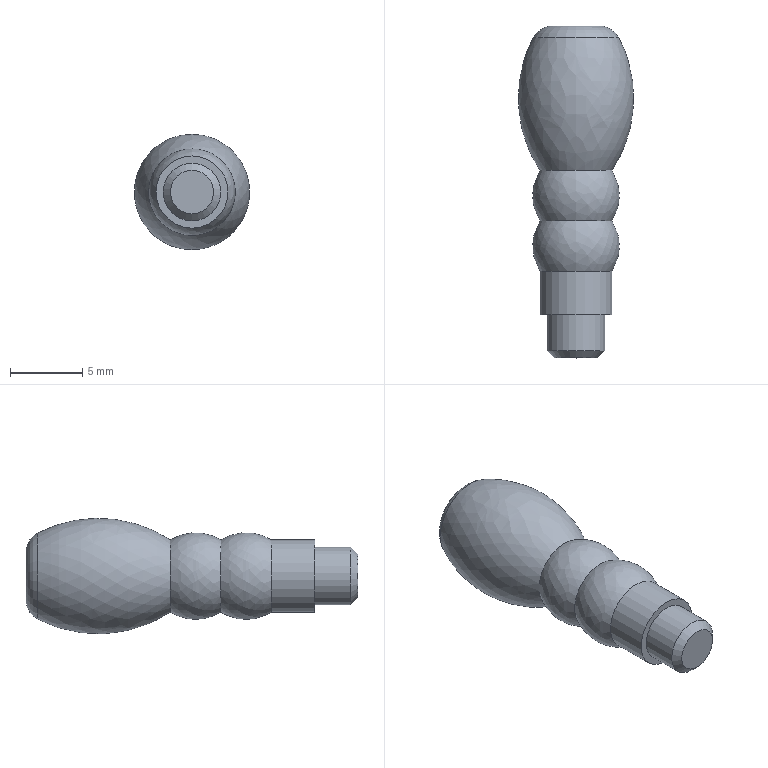Component | NX | 01 | 1 solid | 10 faces | box 8 x 23 x 8 mm | volume 666 mm3 | plane 3 | spline 3 | cylinder 2 | torus 1 | cone 1 | commonest cylinder face diameters 5 x1 4 x1
STEP:
#1=CARTESIAN_POINT('',(0.,0.,0.));
#2=DIRECTION('',(0.,0.,1.));
#3=DIRECTION('',(1.,0.,0.));
#4=AXIS2_PLACEMENT_3D('',#1,#2,#3);
#5=CARTESIAN_POINT('',(0.,-20.,-2.));
#6=VERTEX_POINT('',#5);
#7=CARTESIAN_POINT('',(0.,-20.,0.));
#8=DIRECTION('',(0.,-1.,0.));
#9=DIRECTION('',(0.,0.,-1.));
#10=AXIS2_PLACEMENT_3D('',#7,#8,#9);
#11=CIRCLE('',#10,2.);
#12=CARTESIAN_POINT('',(2.5,-20.,0.));
#13=DIRECTION('',(0.,-1.,0.));
#14=DIRECTION('',(0.,0.,-1.));
#15=AXIS2_PLACEMENT_3D('',#12,#13,#14);
#16=PLANE('',#15);
#17=CARTESIAN_POINT('',(0.,-2.5));
#18=DIRECTION('',(1.,0.));
#19=AXIS2_PLACEMENT_2D('',#17,#18);
#20=CIRCLE('',#19,2.);
#21=(GEOMETRIC_REPRESENTATION_CONTEXT(2)PARAMETRIC_REPRESENTATION_CONTEXT()REPRESENTATION_CONTEXT('',''));
#22=DEFINITIONAL_REPRESENTATION('',(#20),#21);
#23=PCURVE('',#16,#22);
#24=CARTESIAN_POINT('',(0.,-20.,0.));
#25=DIRECTION('',(0.,-1.,0.));
#26=DIRECTION('',(1.,0.,0.));
#27=AXIS2_PLACEMENT_3D('',#24,#25,#26);
#28=CYLINDRICAL_SURFACE('',#27,2.);
#29=CARTESIAN_POINT('',(4.712,0.));
#30=DIRECTION('',(1.,0.));
#31=VECTOR('',#30,1.);
#32=LINE('',#29,#31);
#33=(GEOMETRIC_REPRESENTATION_CONTEXT(2)PARAMETRIC_REPRESENTATION_CONTEXT()REPRESENTATION_CONTEXT('',''));
#34=DEFINITIONAL_REPRESENTATION('',(#32),#33);
#35=PCURVE('',#28,#34);
#36=SURFACE_CURVE('',#11,(#23,#35),.PCURVE_S1.);
#37=EDGE_CURVE('',#6,#6,#36,.T.);
#38=ORIENTED_EDGE('',*,*,#37,.F.);
#39=EDGE_LOOP('',(#38));
#40=FACE_BOUND('',#39,.T.);
#41=CARTESIAN_POINT('',(0.,-20.,2.5));
#42=VERTEX_POINT('',#41);
#43=CARTESIAN_POINT('',(0.,-20.,0.));
#44=DIRECTION('',(0.,1.,0.));
#45=DIRECTION('',(0.,0.,1.));
#46=AXIS2_PLACEMENT_3D('',#43,#44,#45);
#47=CIRCLE('',#46,2.5);
#48=CARTESIAN_POINT('',(-2.5,-2.5));
#49=CARTESIAN_POINT('',(-2.5,1.83));
#50=CARTESIAN_POINT('',(1.25,-0.3349));
#51=CARTESIAN_POINT('',(5.,-2.5));
#52=CARTESIAN_POINT('',(1.25,-4.665));
#53=CARTESIAN_POINT('',(-2.5,-6.83));
#54=CARTESIAN_POINT('',(-2.5,-2.5));
#55=(BOUNDED_CURVE()B_SPLINE_CURVE(2,(#48,#49,#50,#51,#52,#53,#54),.UNSPECIFIED.,.T.,.F.)B_SPLINE_CURVE_WITH_KNOTS((1,2,2,2,2,1),(-2.094,0.,2.094,4.189,6.283,8.378),.UNSPECIFIED.)CURVE()GEOMETRIC_REPRESENTATION_ITEM()RATIONAL_B_SPLINE_CURVE((1.,0.5,1.,0.5,1.,0.5,1.))REPRESENTATION_ITEM(''));
#56=(GEOMETRIC_REPRESENTATION_CONTEXT(2)PARAMETRIC_REPRESENTATION_CONTEXT()REPRESENTATION_CONTEXT('',''));
#57=DEFINITIONAL_REPRESENTATION('',(#55),#56);
#58=PCURVE('',#16,#57);
#59=CARTESIAN_POINT('',(0.,0.,0.));
#60=DIRECTION('',(0.,1.,0.));
#61=DIRECTION('',(0.,0.,1.));
#62=AXIS2_PLACEMENT_3D('',#59,#60,#61);
#63=CYLINDRICAL_SURFACE('',#62,2.5);
#64=CARTESIAN_POINT('',(0.,-20.));
#65=DIRECTION('',(1.,0.));
#66=VECTOR('',#65,1.);
#67=LINE('',#64,#66);
#68=(GEOMETRIC_REPRESENTATION_CONTEXT(2)PARAMETRIC_REPRESENTATION_CONTEXT()REPRESENTATION_CONTEXT('',''));
#69=DEFINITIONAL_REPRESENTATION('',(#67),#68);
#70=PCURVE('',#63,#69);
#71=SURFACE_CURVE('',#47,(#58,#70),.PCURVE_S1.);
#72=EDGE_CURVE('',#42,#42,#71,.T.);
#73=ORIENTED_EDGE('',*,*,#72,.F.);
#74=EDGE_LOOP('',(#73));
#75=FACE_BOUND('',#74,.T.);
#76=ADVANCED_FACE('',(#40,#75),#16,.T.);
#77=ORIENTED_EDGE('',*,*,#72,.T.);
#78=CARTESIAN_POINT('',(0.,-17.,2.5));
#79=VERTEX_POINT('',#78);
#80=CARTESIAN_POINT('',(0.,-20.,2.5));
#81=CARTESIAN_POINT('',(0.,-17.,2.5));
#82=B_SPLINE_CURVE_WITH_KNOTS('',1,(#80,#81),.UNSPECIFIED.,.F.,.F.,(2,2),(-20.,-17.),.PIECEWISE_BEZIER_KNOTS.);
#83=CARTESIAN_POINT('',(6.283,0.));
#84=DIRECTION('',(0.,1.));
#85=VECTOR('',#84,1.);
#86=LINE('',#83,#85);
#87=(GEOMETRIC_REPRESENTATION_CONTEXT(2)PARAMETRIC_REPRESENTATION_CONTEXT()REPRESENTATION_CONTEXT('',''));
#88=DEFINITIONAL_REPRESENTATION('',(#86),#87);
#89=PCURVE('',#63,#88);
#90=CARTESIAN_POINT('',(0.,0.));
#91=DIRECTION('',(0.,1.));
#92=VECTOR('',#91,1.);
#93=LINE('',#90,#92);
#94=(GEOMETRIC_REPRESENTATION_CONTEXT(2)PARAMETRIC_REPRESENTATION_CONTEXT()REPRESENTATION_CONTEXT('',''));
#95=DEFINITIONAL_REPRESENTATION('',(#93),#94);
#96=PCURVE('',#63,#95);
#97=SEAM_CURVE('',#82,(#89,#96),.PCURVE_S1.);
#98=EDGE_CURVE('',#42,#79,#97,.T.);
#99=ORIENTED_EDGE('',*,*,#98,.T.);
#100=CARTESIAN_POINT('',(0.,-17.,0.));
#101=DIRECTION('',(0.,1.,0.));
#102=DIRECTION('',(0.,0.,1.));
#103=AXIS2_PLACEMENT_3D('',#100,#101,#102);
#104=CIRCLE('',#103,2.5);
#105=CARTESIAN_POINT('',(0.,-17.));
#106=DIRECTION('',(1.,0.));
#107=VECTOR('',#106,1.);
#108=LINE('',#105,#107);
#109=(GEOMETRIC_REPRESENTATION_CONTEXT(2)PARAMETRIC_REPRESENTATION_CONTEXT()REPRESENTATION_CONTEXT('',''));
#110=DEFINITIONAL_REPRESENTATION('',(#108),#109);
#111=PCURVE('',#63,#110);
#112=CARTESIAN_POINT('',(0.,-13.5,2.5));
#113=CARTESIAN_POINT('',(5.,-13.5,2.5));
#114=CARTESIAN_POINT('',(5.,-13.5,-2.5));
#115=CARTESIAN_POINT('',(0.,-13.5,-2.5));
#116=CARTESIAN_POINT('',(-5.,-13.5,-2.5));
#117=CARTESIAN_POINT('',(-5.,-13.5,2.5));
#118=CARTESIAN_POINT('',(0.,-13.5,2.5));
#119=CARTESIAN_POINT('',(0.,-14.601,3.185));
#120=CARTESIAN_POINT('',(6.371,-14.601,3.185));
#121=CARTESIAN_POINT('',(6.371,-14.601,-3.185));
#122=CARTESIAN_POINT('',(0.,-14.601,-3.185));
#123=CARTESIAN_POINT('',(-6.371,-14.601,-3.185));
#124=CARTESIAN_POINT('',(-6.371,-14.601,3.185));
#125=CARTESIAN_POINT('',(0.,-14.601,3.185));
#126=CARTESIAN_POINT('',(0.,-15.899,3.185));
#127=CARTESIAN_POINT('',(6.371,-15.899,3.185));
#128=CARTESIAN_POINT('',(6.371,-15.899,-3.185));
#129=CARTESIAN_POINT('',(0.,-15.899,-3.185));
#130=CARTESIAN_POINT('',(-6.371,-15.899,-3.185));
#131=CARTESIAN_POINT('',(-6.371,-15.899,3.185));
#132=CARTESIAN_POINT('',(0.,-15.899,3.185));
#133=CARTESIAN_POINT('',(0.,-17.,2.5));
#134=CARTESIAN_POINT('',(5.,-17.,2.5));
#135=CARTESIAN_POINT('',(5.,-17.,-2.5));
#136=CARTESIAN_POINT('',(0.,-17.,-2.5));
#137=CARTESIAN_POINT('',(-5.,-17.,-2.5));
#138=CARTESIAN_POINT('',(-5.,-17.,2.5));
#139=CARTESIAN_POINT('',(0.,-17.,2.5));
#140=(BOUNDED_SURFACE()B_SPLINE_SURFACE(3,3,((#112,#113,#114,#115,#116,#117,#118),(#119,#120,#121,#122,#123,#124,#125),(#126,#127,#128,#129,#130,#131,#132),(#133,#134,#135,#136,#137,#138,#139)),.UNSPECIFIED.,.F.,.T.,.F.)B_SPLINE_SURFACE_WITH_KNOTS((4,4),(1,3,3,3,1),(0.,1.),(-0.5,0.,0.5,1.,1.5),.UNSPECIFIED.)GEOMETRIC_REPRESENTATION_ITEM()RATIONAL_B_SPLINE_SURFACE(((1.,0.3333,0.3333,1.,0.3333,0.3333,1.),(0.8994,0.2998,0.2998,0.8994,0.2998,0.2998,0.8994),(0.8994,0.2998,0.2998,0.8994,0.2998,0.2998,0.8994),(1.,0.3333,0.3333,1.,0.3333,0.3333,1.)))REPRESENTATION_ITEM('')SURFACE());
#141=CARTESIAN_POINT('',(1.,0.));
#142=CARTESIAN_POINT('',(1.,0.02352));
#143=CARTESIAN_POINT('',(1.,0.06491));
#144=CARTESIAN_POINT('',(1.,0.1146));
#145=CARTESIAN_POINT('',(1.,0.1575));
#146=CARTESIAN_POINT('',(1.,0.196));
#147=CARTESIAN_POINT('',(1.,0.2322));
#148=CARTESIAN_POINT('',(1.,0.2678));
#149=CARTESIAN_POINT('',(1.,0.304));
#150=CARTESIAN_POINT('',(1.,0.3425));
#151=CARTESIAN_POINT('',(1.,0.3856));
#152=CARTESIAN_POINT('',(1.,0.4343));
#153=CARTESIAN_POINT('',(1.,0.5));
#154=CARTESIAN_POINT('',(1.,0.5657));
#155=CARTESIAN_POINT('',(1.,0.6144));
#156=CARTESIAN_POINT('',(1.,0.6575));
#157=CARTESIAN_POINT('',(1.,0.696));
#158=CARTESIAN_POINT('',(1.,0.7322));
#159=CARTESIAN_POINT('',(1.,0.7678));
#160=CARTESIAN_POINT('',(1.,0.804));
#161=CARTESIAN_POINT('',(1.,0.8425));
#162=CARTESIAN_POINT('',(1.,0.8854));
#163=CARTESIAN_POINT('',(1.,0.9351));
#164=CARTESIAN_POINT('',(1.,0.9765));
#165=CARTESIAN_POINT('',(1.,1.));
#166=B_SPLINE_CURVE_WITH_KNOTS('',3,(#141,#142,#143,#144,#145,#146,#147,#148,#149,#150,#151,#152,#153,#154,#155,#156,#157,#158,#159,#160,#161,#162,#163,#164,#165),.UNSPECIFIED.,.F.,.F.,(4,1,1,1,1,1,1,1,1,1,1,1,1,1,1,1,1,1,1,1,1,1,4),(0.,0.2856,0.5712,0.8568,1.142,1.428,1.714,1.999,2.285,2.57,2.856,3.142,3.427,3.713,3.998,4.284,4.57,4.855,5.141,5.426,5.712,5.998,6.283),.QUASI_UNIFORM_KNOTS.);
#167=(GEOMETRIC_REPRESENTATION_CONTEXT(2)PARAMETRIC_REPRESENTATION_CONTEXT()REPRESENTATION_CONTEXT('',''));
#168=DEFINITIONAL_REPRESENTATION('',(#166),#167);
#169=PCURVE('',#140,#168);
#170=SURFACE_CURVE('',#104,(#111,#169),.PCURVE_S1.);
#171=EDGE_CURVE('',#79,#79,#170,.T.);
#172=ORIENTED_EDGE('',*,*,#171,.F.);
#173=ORIENTED_EDGE('',*,*,#98,.F.);
#174=EDGE_LOOP('',(#77,#99,#172,#173));
#175=FACE_BOUND('',#174,.T.);
#176=ADVANCED_FACE('',(#175),#63,.T.);
#177=ORIENTED_EDGE('',*,*,#171,.T.);
#178=CARTESIAN_POINT('',(0.,-13.5,2.5));
#179=VERTEX_POINT('',#178);
#180=CARTESIAN_POINT('',(0.,-13.5,2.5));
#181=CARTESIAN_POINT('',(0.,-14.601,3.185));
#182=CARTESIAN_POINT('',(0.,-15.899,3.185));
#183=CARTESIAN_POINT('',(0.,-17.,2.5));
#184=(BOUNDED_CURVE()B_SPLINE_CURVE(3,(#180,#181,#182,#183),.UNSPECIFIED.,.F.,.F.)B_SPLINE_CURVE_WITH_KNOTS((4,4),(0.,1.),.PIECEWISE_BEZIER_KNOTS.)CURVE()GEOMETRIC_REPRESENTATION_ITEM()RATIONAL_B_SPLINE_CURVE((1.,0.8994,0.8994,1.))REPRESENTATION_ITEM(''));
#185=CARTESIAN_POINT('',(0.,1.));
#186=DIRECTION('',(1.,0.));
#187=VECTOR('',#186,1.);
#188=LINE('',#185,#187);
#189=(GEOMETRIC_REPRESENTATION_CONTEXT(2)PARAMETRIC_REPRESENTATION_CONTEXT()REPRESENTATION_CONTEXT('',''));
#190=DEFINITIONAL_REPRESENTATION('',(#188),#189);
#191=PCURVE('',#140,#190);
#192=CARTESIAN_POINT('',(0.,0.));
#193=DIRECTION('',(1.,0.));
#194=VECTOR('',#193,1.);
#195=LINE('',#192,#194);
#196=(GEOMETRIC_REPRESENTATION_CONTEXT(2)PARAMETRIC_REPRESENTATION_CONTEXT()REPRESENTATION_CONTEXT('',''));
#197=DEFINITIONAL_REPRESENTATION('',(#195),#196);
#198=PCURVE('',#140,#197);
#199=SEAM_CURVE('',#184,(#191,#198),.PCURVE_S1.);
#200=EDGE_CURVE('',#179,#79,#199,.T.);
#201=ORIENTED_EDGE('',*,*,#200,.F.);
#202=CARTESIAN_POINT('',(0.,-13.5,0.));
#203=DIRECTION('',(0.,1.,0.));
#204=DIRECTION('',(0.,0.,1.));
#205=AXIS2_PLACEMENT_3D('',#202,#203,#204);
#206=CIRCLE('',#205,2.5);
#207=CARTESIAN_POINT('',(0.,0.));
#208=CARTESIAN_POINT('',(0.,0.02352));
#209=CARTESIAN_POINT('',(0.,0.06491));
#210=CARTESIAN_POINT('',(0.,0.1146));
#211=CARTESIAN_POINT('',(0.,0.1575));
#212=CARTESIAN_POINT('',(0.,0.196));
#213=CARTESIAN_POINT('',(0.,0.2322));
#214=CARTESIAN_POINT('',(0.,0.2678));
#215=CARTESIAN_POINT('',(0.,0.304));
#216=CARTESIAN_POINT('',(0.,0.3425));
#217=CARTESIAN_POINT('',(0.,0.3856));
#218=CARTESIAN_POINT('',(0.,0.4343));
#219=CARTESIAN_POINT('',(0.,0.5));
#220=CARTESIAN_POINT('',(0.,0.5657));
#221=CARTESIAN_POINT('',(0.,0.6144));
#222=CARTESIAN_POINT('',(0.,0.6575));
#223=CARTESIAN_POINT('',(0.,0.696));
#224=CARTESIAN_POINT('',(0.,0.7322));
#225=CARTESIAN_POINT('',(0.,0.7678));
#226=CARTESIAN_POINT('',(0.,0.804));
#227=CARTESIAN_POINT('',(0.,0.8425));
#228=CARTESIAN_POINT('',(0.,0.8854));
#229=CARTESIAN_POINT('',(0.,0.9351));
#230=CARTESIAN_POINT('',(0.,0.9765));
#231=CARTESIAN_POINT('',(0.,1.));
#232=B_SPLINE_CURVE_WITH_KNOTS('',3,(#207,#208,#209,#210,#211,#212,#213,#214,#215,#216,#217,#218,#219,#220,#221,#222,#223,#224,#225,#226,#227,#228,#229,#230,#231),.UNSPECIFIED.,.F.,.F.,(4,1,1,1,1,1,1,1,1,1,1,1,1,1,1,1,1,1,1,1,1,1,4),(0.,0.2856,0.5712,0.8568,1.142,1.428,1.714,1.999,2.285,2.57,2.856,3.142,3.427,3.713,3.998,4.284,4.57,4.855,5.141,5.426,5.712,5.998,6.283),.QUASI_UNIFORM_KNOTS.);
#233=(GEOMETRIC_REPRESENTATION_CONTEXT(2)PARAMETRIC_REPRESENTATION_CONTEXT()REPRESENTATION_CONTEXT('',''));
#234=DEFINITIONAL_REPRESENTATION('',(#232),#233);
#235=PCURVE('',#140,#234);
#236=CARTESIAN_POINT('',(0.,-10.,2.5));
#237=CARTESIAN_POINT('',(5.,-10.,2.5));
#238=CARTESIAN_POINT('',(5.,-10.,-2.5));
#239=CARTESIAN_POINT('',(0.,-10.,-2.5));
#240=CARTESIAN_POINT('',(-5.,-10.,-2.5));
#241=CARTESIAN_POINT('',(-5.,-10.,2.5));
#242=CARTESIAN_POINT('',(0.,-10.,2.5));
#243=CARTESIAN_POINT('',(0.,-11.101,3.185));
#244=CARTESIAN_POINT('',(6.371,-11.101,3.185));
#245=CARTESIAN_POINT('',(6.371,-11.101,-3.185));
#246=CARTESIAN_POINT('',(0.,-11.101,-3.185));
#247=CARTESIAN_POINT('',(-6.371,-11.101,-3.185));
#248=CARTESIAN_POINT('',(-6.371,-11.101,3.185));
#249=CARTESIAN_POINT('',(0.,-11.101,3.185));
#250=CARTESIAN_POINT('',(0.,-12.399,3.185));
#251=CARTESIAN_POINT('',(6.371,-12.399,3.185));
#252=CARTESIAN_POINT('',(6.371,-12.399,-3.185));
#253=CARTESIAN_POINT('',(0.,-12.399,-3.185));
#254=CARTESIAN_POINT('',(-6.371,-12.399,-3.185));
#255=CARTESIAN_POINT('',(-6.371,-12.399,3.185));
#256=CARTESIAN_POINT('',(0.,-12.399,3.185));
#257=CARTESIAN_POINT('',(0.,-13.5,2.5));
#258=CARTESIAN_POINT('',(5.,-13.5,2.5));
#259=CARTESIAN_POINT('',(5.,-13.5,-2.5));
#260=CARTESIAN_POINT('',(0.,-13.5,-2.5));
#261=CARTESIAN_POINT('',(-5.,-13.5,-2.5));
#262=CARTESIAN_POINT('',(-5.,-13.5,2.5));
#263=CARTESIAN_POINT('',(0.,-13.5,2.5));
#264=(BOUNDED_SURFACE()B_SPLINE_SURFACE(3,3,((#236,#237,#238,#239,#240,#241,#242),(#243,#244,#245,#246,#247,#248,#249),(#250,#251,#252,#253,#254,#255,#256),(#257,#258,#259,#260,#261,#262,#263)),.UNSPECIFIED.,.F.,.T.,.F.)B_SPLINE_SURFACE_WITH_KNOTS((4,4),(1,3,3,3,1),(0.,1.),(-0.5,0.,0.5,1.,1.5),.UNSPECIFIED.)GEOMETRIC_REPRESENTATION_ITEM()RATIONAL_B_SPLINE_SURFACE(((1.,0.3333,0.3333,1.,0.3333,0.3333,1.),(0.8994,0.2998,0.2998,0.8994,0.2998,0.2998,0.8994),(0.8994,0.2998,0.2998,0.8994,0.2998,0.2998,0.8994),(1.,0.3333,0.3333,1.,0.3333,0.3333,1.)))REPRESENTATION_ITEM('')SURFACE());
#265=CARTESIAN_POINT('',(1.,0.));
#266=CARTESIAN_POINT('',(1.,0.02352));
#267=CARTESIAN_POINT('',(1.,0.06491));
#268=CARTESIAN_POINT('',(1.,0.1146));
#269=CARTESIAN_POINT('',(1.,0.1575));
#270=CARTESIAN_POINT('',(1.,0.196));
#271=CARTESIAN_POINT('',(1.,0.2322));
#272=CARTESIAN_POINT('',(1.,0.2678));
#273=CARTESIAN_POINT('',(1.,0.304));
#274=CARTESIAN_POINT('',(1.,0.3425));
#275=CARTESIAN_POINT('',(1.,0.3856));
#276=CARTESIAN_POINT('',(1.,0.4343));
#277=CARTESIAN_POINT('',(1.,0.5));
#278=CARTESIAN_POINT('',(1.,0.5657));
#279=CARTESIAN_POINT('',(1.,0.6144));
#280=CARTESIAN_POINT('',(1.,0.6575));
#281=CARTESIAN_POINT('',(1.,0.696));
#282=CARTESIAN_POINT('',(1.,0.7322));
#283=CARTESIAN_POINT('',(1.,0.7678));
#284=CARTESIAN_POINT('',(1.,0.804));
#285=CARTESIAN_POINT('',(1.,0.8425));
#286=CARTESIAN_POINT('',(1.,0.8854));
#287=CARTESIAN_POINT('',(1.,0.9351));
#288=CARTESIAN_POINT('',(1.,0.9765));
#289=CARTESIAN_POINT('',(1.,1.));
#290=B_SPLINE_CURVE_WITH_KNOTS('',3,(#265,#266,#267,#268,#269,#270,#271,#272,#273,#274,#275,#276,#277,#278,#279,#280,#281,#282,#283,#284,#285,#286,#287,#288,#289),.UNSPECIFIED.,.F.,.F.,(4,1,1,1,1,1,1,1,1,1,1,1,1,1,1,1,1,1,1,1,1,1,4),(0.,0.2856,0.5712,0.8568,1.142,1.428,1.714,1.999,2.285,2.57,2.856,3.142,3.427,3.713,3.998,4.284,4.57,4.855,5.141,5.426,5.712,5.998,6.283),.QUASI_UNIFORM_KNOTS.);
#291=(GEOMETRIC_REPRESENTATION_CONTEXT(2)PARAMETRIC_REPRESENTATION_CONTEXT()REPRESENTATION_CONTEXT('',''));
#292=DEFINITIONAL_REPRESENTATION('',(#290),#291);
#293=PCURVE('',#264,#292);
#294=SURFACE_CURVE('',#206,(#235,#293),.PCURVE_S1.);
#295=EDGE_CURVE('',#179,#179,#294,.T.);
#296=ORIENTED_EDGE('',*,*,#295,.F.);
#297=ORIENTED_EDGE('',*,*,#200,.T.);
#298=EDGE_LOOP('',(#177,#201,#296,#297));
#299=FACE_BOUND('',#298,.T.);
#300=ADVANCED_FACE('',(#299),#140,.T.);
#301=ORIENTED_EDGE('',*,*,#295,.T.);
#302=CARTESIAN_POINT('',(0.,-10.,2.5));
#303=VERTEX_POINT('',#302);
#304=CARTESIAN_POINT('',(0.,-10.,2.5));
#305=CARTESIAN_POINT('',(0.,-11.101,3.185));
#306=CARTESIAN_POINT('',(0.,-12.399,3.185));
#307=CARTESIAN_POINT('',(0.,-13.5,2.5));
#308=(BOUNDED_CURVE()B_SPLINE_CURVE(3,(#304,#305,#306,#307),.UNSPECIFIED.,.F.,.F.)B_SPLINE_CURVE_WITH_KNOTS((4,4),(0.,1.),.PIECEWISE_BEZIER_KNOTS.)CURVE()GEOMETRIC_REPRESENTATION_ITEM()RATIONAL_B_SPLINE_CURVE((1.,0.8994,0.8994,1.))REPRESENTATION_ITEM(''));
#309=CARTESIAN_POINT('',(0.,1.));
#310=DIRECTION('',(1.,0.));
#311=VECTOR('',#310,1.);
#312=LINE('',#309,#311);
#313=(GEOMETRIC_REPRESENTATION_CONTEXT(2)PARAMETRIC_REPRESENTATION_CONTEXT()REPRESENTATION_CONTEXT('',''));
#314=DEFINITIONAL_REPRESENTATION('',(#312),#313);
#315=PCURVE('',#264,#314);
#316=CARTESIAN_POINT('',(0.,0.));
#317=DIRECTION('',(1.,0.));
#318=VECTOR('',#317,1.);
#319=LINE('',#316,#318);
#320=(GEOMETRIC_REPRESENTATION_CONTEXT(2)PARAMETRIC_REPRESENTATION_CONTEXT()REPRESENTATION_CONTEXT('',''));
#321=DEFINITIONAL_REPRESENTATION('',(#319),#320);
#322=PCURVE('',#264,#321);
#323=SEAM_CURVE('',#308,(#315,#322),.PCURVE_S1.);
#324=EDGE_CURVE('',#303,#179,#323,.T.);
#325=ORIENTED_EDGE('',*,*,#324,.F.);
#326=CARTESIAN_POINT('',(0.,-10.,0.));
#327=DIRECTION('',(0.,1.,0.));
#328=DIRECTION('',(0.,0.,1.));
#329=AXIS2_PLACEMENT_3D('',#326,#327,#328);
#330=CIRCLE('',#329,2.5);
#331=CARTESIAN_POINT('',(0.,0.));
#332=CARTESIAN_POINT('',(0.,0.02352));
#333=CARTESIAN_POINT('',(0.,0.06491));
#334=CARTESIAN_POINT('',(0.,0.1146));
#335=CARTESIAN_POINT('',(0.,0.1575));
#336=CARTESIAN_POINT('',(0.,0.196));
#337=CARTESIAN_POINT('',(0.,0.2322));
#338=CARTESIAN_POINT('',(0.,0.2678));
#339=CARTESIAN_POINT('',(0.,0.304));
#340=CARTESIAN_POINT('',(0.,0.3425));
#341=CARTESIAN_POINT('',(0.,0.3856));
#342=CARTESIAN_POINT('',(0.,0.4343));
#343=CARTESIAN_POINT('',(0.,0.5));
#344=CARTESIAN_POINT('',(0.,0.5657));
#345=CARTESIAN_POINT('',(0.,0.6144));
#346=CARTESIAN_POINT('',(0.,0.6575));
#347=CARTESIAN_POINT('',(0.,0.696));
#348=CARTESIAN_POINT('',(0.,0.7322));
#349=CARTESIAN_POINT('',(0.,0.7678));
#350=CARTESIAN_POINT('',(0.,0.804));
#351=CARTESIAN_POINT('',(0.,0.8425));
#352=CARTESIAN_POINT('',(0.,0.8854));
#353=CARTESIAN_POINT('',(0.,0.9351));
#354=CARTESIAN_POINT('',(0.,0.9765));
#355=CARTESIAN_POINT('',(0.,1.));
#356=B_SPLINE_CURVE_WITH_KNOTS('',3,(#331,#332,#333,#334,#335,#336,#337,#338,#339,#340,#341,#342,#343,#344,#345,#346,#347,#348,#349,#350,#351,#352,#353,#354,#355),.UNSPECIFIED.,.F.,.F.,(4,1,1,1,1,1,1,1,1,1,1,1,1,1,1,1,1,1,1,1,1,1,4),(0.,0.2856,0.5712,0.8568,1.142,1.428,1.714,1.999,2.285,2.57,2.856,3.142,3.427,3.713,3.998,4.284,4.57,4.855,5.141,5.426,5.712,5.998,6.283),.QUASI_UNIFORM_KNOTS.);
#357=(GEOMETRIC_REPRESENTATION_CONTEXT(2)PARAMETRIC_REPRESENTATION_CONTEXT()REPRESENTATION_CONTEXT('',''));
#358=DEFINITIONAL_REPRESENTATION('',(#356),#357);
#359=PCURVE('',#264,#358);
#360=CARTESIAN_POINT('',(0.,-0.8077,2.975));
#361=CARTESIAN_POINT('',(5.949,-0.8077,2.975));
#362=CARTESIAN_POINT('',(5.949,-0.8077,-2.975));
#363=CARTESIAN_POINT('',(0.,-0.8077,-2.975));
#364=CARTESIAN_POINT('',(-5.949,-0.8077,-2.975));
#365=CARTESIAN_POINT('',(-5.949,-0.8077,2.975));
#366=CARTESIAN_POINT('',(0.,-0.8077,2.975));
#367=CARTESIAN_POINT('',(0.,-3.805,4.534));
#368=CARTESIAN_POINT('',(9.068,-3.805,4.534));
#369=CARTESIAN_POINT('',(9.068,-3.805,-4.534));
#370=CARTESIAN_POINT('',(0.,-3.805,-4.534));
#371=CARTESIAN_POINT('',(-9.068,-3.805,-4.534));
#372=CARTESIAN_POINT('',(-9.068,-3.805,4.534));
#373=CARTESIAN_POINT('',(0.,-3.805,4.534));
#374=CARTESIAN_POINT('',(0.,-7.179,4.36));
#375=CARTESIAN_POINT('',(8.72,-7.179,4.36));
#376=CARTESIAN_POINT('',(8.72,-7.179,-4.36));
#377=CARTESIAN_POINT('',(0.,-7.179,-4.36));
#378=CARTESIAN_POINT('',(-8.72,-7.179,-4.36));
#379=CARTESIAN_POINT('',(-8.72,-7.179,4.36));
#380=CARTESIAN_POINT('',(0.,-7.179,4.36));
#381=CARTESIAN_POINT('',(0.,-10.,2.5));
#382=CARTESIAN_POINT('',(5.,-10.,2.5));
#383=CARTESIAN_POINT('',(5.,-10.,-2.5));
#384=CARTESIAN_POINT('',(0.,-10.,-2.5));
#385=CARTESIAN_POINT('',(-5.,-10.,-2.5));
#386=CARTESIAN_POINT('',(-5.,-10.,2.5));
#387=CARTESIAN_POINT('',(0.,-10.,2.5));
#388=(BOUNDED_SURFACE()B_SPLINE_SURFACE(3,3,((#360,#361,#362,#363,#364,#365,#366),(#367,#368,#369,#370,#371,#372,#373),(#374,#375,#376,#377,#378,#379,#380),(#381,#382,#383,#384,#385,#386,#387)),.UNSPECIFIED.,.F.,.T.,.F.)B_SPLINE_SURFACE_WITH_KNOTS((4,4),(1,3,3,3,1),(0.,1.),(-0.5,0.,0.5,1.,1.5),.UNSPECIFIED.)GEOMETRIC_REPRESENTATION_ITEM()RATIONAL_B_SPLINE_SURFACE(((1.,0.3333,0.3333,1.,0.3333,0.3333,1.),(0.9081,0.3027,0.3027,0.9081,0.3027,0.3027,0.9081),(0.9081,0.3027,0.3027,0.9081,0.3027,0.3027,0.9081),(1.,0.3333,0.3333,1.,0.3333,0.3333,1.)))REPRESENTATION_ITEM('')SURFACE());
#389=CARTESIAN_POINT('',(1.,0.));
#390=CARTESIAN_POINT('',(1.,0.02352));
#391=CARTESIAN_POINT('',(1.,0.06491));
#392=CARTESIAN_POINT('',(1.,0.1146));
#393=CARTESIAN_POINT('',(1.,0.1575));
#394=CARTESIAN_POINT('',(1.,0.196));
#395=CARTESIAN_POINT('',(1.,0.2322));
#396=CARTESIAN_POINT('',(1.,0.2678));
#397=CARTESIAN_POINT('',(1.,0.304));
#398=CARTESIAN_POINT('',(1.,0.3425));
#399=CARTESIAN_POINT('',(1.,0.3856));
#400=CARTESIAN_POINT('',(1.,0.4343));
#401=CARTESIAN_POINT('',(1.,0.5));
#402=CARTESIAN_POINT('',(1.,0.5657));
#403=CARTESIAN_POINT('',(1.,0.6144));
#404=CARTESIAN_POINT('',(1.,0.6575));
#405=CARTESIAN_POINT('',(1.,0.696));
#406=CARTESIAN_POINT('',(1.,0.7322));
#407=CARTESIAN_POINT('',(1.,0.7678));
#408=CARTESIAN_POINT('',(1.,0.804));
#409=CARTESIAN_POINT('',(1.,0.8425));
#410=CARTESIAN_POINT('',(1.,0.8854));
#411=CARTESIAN_POINT('',(1.,0.9351));
#412=CARTESIAN_POINT('',(1.,0.9765));
#413=CARTESIAN_POINT('',(1.,1.));
#414=B_SPLINE_CURVE_WITH_KNOTS('',3,(#389,#390,#391,#392,#393,#394,#395,#396,#397,#398,#399,#400,#401,#402,#403,#404,#405,#406,#407,#408,#409,#410,#411,#412,#413),.UNSPECIFIED.,.F.,.F.,(4,1,1,1,1,1,1,1,1,1,1,1,1,1,1,1,1,1,1,1,1,1,4),(0.,0.2856,0.5712,0.8568,1.142,1.428,1.714,1.999,2.285,2.57,2.856,3.142,3.427,3.713,3.998,4.284,4.57,4.855,5.141,5.426,5.712,5.998,6.283),.QUASI_UNIFORM_KNOTS.);
#415=(GEOMETRIC_REPRESENTATION_CONTEXT(2)PARAMETRIC_REPRESENTATION_CONTEXT()REPRESENTATION_CONTEXT('',''));
#416=DEFINITIONAL_REPRESENTATION('',(#414),#415);
#417=PCURVE('',#388,#416);
#418=SURFACE_CURVE('',#330,(#359,#417),.PCURVE_S1.);
#419=EDGE_CURVE('',#303,#303,#418,.T.);
#420=ORIENTED_EDGE('',*,*,#419,.F.);
#421=ORIENTED_EDGE('',*,*,#324,.T.);
#422=EDGE_LOOP('',(#301,#325,#420,#421));
#423=FACE_BOUND('',#422,.T.);
#424=ADVANCED_FACE('',(#423),#264,.T.);
#425=CARTESIAN_POINT('',(0.,-0.8077,-2.975));
#426=VERTEX_POINT('',#425);
#427=CARTESIAN_POINT('',(0.,-0.8077,2.975));
#428=VERTEX_POINT('',#427);
#429=CARTESIAN_POINT('',(0.,-0.8077,0.));
#430=DIRECTION('',(0.,-1.,0.));
#431=DIRECTION('',(0.,0.,-1.));
#432=AXIS2_PLACEMENT_3D('',#429,#430,#431);
#433=CIRCLE('',#432,2.975);
#434=CARTESIAN_POINT('',(0.,0.5));
#435=CARTESIAN_POINT('',(0.,0.4765));
#436=CARTESIAN_POINT('',(0.,0.4351));
#437=CARTESIAN_POINT('',(0.,0.3854));
#438=CARTESIAN_POINT('',(0.,0.3425));
#439=CARTESIAN_POINT('',(0.,0.304));
#440=CARTESIAN_POINT('',(0.,0.2678));
#441=CARTESIAN_POINT('',(0.,0.2322));
#442=CARTESIAN_POINT('',(0.,0.196));
#443=CARTESIAN_POINT('',(0.,0.1575));
#444=CARTESIAN_POINT('',(0.,0.1144));
#445=CARTESIAN_POINT('',(0.,0.06567));
#446=CARTESIAN_POINT('',(0.,0.));
#447=CARTESIAN_POINT('',(0.,-0.06567));
#448=CARTESIAN_POINT('',(0.,-0.1144));
#449=CARTESIAN_POINT('',(0.,-0.1575));
#450=CARTESIAN_POINT('',(0.,-0.196));
#451=CARTESIAN_POINT('',(0.,-0.2322));
#452=CARTESIAN_POINT('',(0.,-0.2678));
#453=CARTESIAN_POINT('',(0.,-0.304));
#454=CARTESIAN_POINT('',(0.,-0.3425));
#455=CARTESIAN_POINT('',(0.,-0.3854));
#456=CARTESIAN_POINT('',(0.,-0.4351));
#457=CARTESIAN_POINT('',(0.,-0.4765));
#458=CARTESIAN_POINT('',(0.,-0.5));
#459=B_SPLINE_CURVE_WITH_KNOTS('',3,(#434,#435,#436,#437,#438,#439,#440,#441,#442,#443,#444,#445,#446,#447,#448,#449,#450,#451,#452,#453,#454,#455,#456,#457,#458),.UNSPECIFIED.,.F.,.F.,(4,1,1,1,1,1,1,1,1,1,1,1,1,1,1,1,1,1,1,1,1,1,4),(0.,0.2856,0.5712,0.8568,1.142,1.428,1.714,1.999,2.285,2.57,2.856,3.142,3.427,3.713,3.998,4.284,4.57,4.855,5.141,5.426,5.712,5.998,6.283),.QUASI_UNIFORM_KNOTS.);
#460=(GEOMETRIC_REPRESENTATION_CONTEXT(2)PARAMETRIC_REPRESENTATION_CONTEXT()REPRESENTATION_CONTEXT('',''));
#461=DEFINITIONAL_REPRESENTATION('',(#459),#460);
#462=PCURVE('',#388,#461);
#463=CARTESIAN_POINT('',(0.,-1.5,0.));
#464=DIRECTION('',(0.,1.,0.));
#465=DIRECTION('',(0.,0.,1.));
#466=AXIS2_PLACEMENT_3D('',#463,#464,#465);
#467=TOROIDAL_SURFACE('',#466,1.644,1.5);
#468=CARTESIAN_POINT('',(3.142,6.763));
#469=DIRECTION('',(-1.,0.));
#470=VECTOR('',#469,1.);
#471=LINE('',#468,#470);
#472=(GEOMETRIC_REPRESENTATION_CONTEXT(2)PARAMETRIC_REPRESENTATION_CONTEXT()REPRESENTATION_CONTEXT('',''));
#473=DEFINITIONAL_REPRESENTATION('',(#471),#472);
#474=PCURVE('',#467,#473);
#475=SURFACE_CURVE('',#433,(#462,#474),.PCURVE_S1.);
#476=EDGE_CURVE('',#426,#428,#475,.T.);
#477=ORIENTED_EDGE('',*,*,#476,.T.);
#478=CARTESIAN_POINT('',(0.,-0.8077,2.975));
#479=CARTESIAN_POINT('',(0.,-3.805,4.534));
#480=CARTESIAN_POINT('',(0.,-7.179,4.36));
#481=CARTESIAN_POINT('',(0.,-10.,2.5));
#482=(BOUNDED_CURVE()B_SPLINE_CURVE(3,(#478,#479,#480,#481),.UNSPECIFIED.,.F.,.F.)B_SPLINE_CURVE_WITH_KNOTS((4,4),(0.,1.),.PIECEWISE_BEZIER_KNOTS.)CURVE()GEOMETRIC_REPRESENTATION_ITEM()RATIONAL_B_SPLINE_CURVE((1.,0.9081,0.9081,1.))REPRESENTATION_ITEM(''));
#483=CARTESIAN_POINT('',(0.,0.));
#484=DIRECTION('',(1.,0.));
#485=VECTOR('',#484,1.);
#486=LINE('',#483,#485);
#487=(GEOMETRIC_REPRESENTATION_CONTEXT(2)PARAMETRIC_REPRESENTATION_CONTEXT()REPRESENTATION_CONTEXT('',''));
#488=DEFINITIONAL_REPRESENTATION('',(#486),#487);
#489=PCURVE('',#388,#488);
#490=CARTESIAN_POINT('',(0.,1.));
#491=DIRECTION('',(1.,0.));
#492=VECTOR('',#491,1.);
#493=LINE('',#490,#492);
#494=(GEOMETRIC_REPRESENTATION_CONTEXT(2)PARAMETRIC_REPRESENTATION_CONTEXT()REPRESENTATION_CONTEXT('',''));
#495=DEFINITIONAL_REPRESENTATION('',(#493),#494);
#496=PCURVE('',#388,#495);
#497=SEAM_CURVE('',#482,(#489,#496),.PCURVE_S1.);
#498=EDGE_CURVE('',#428,#303,#497,.T.);
#499=ORIENTED_EDGE('',*,*,#498,.T.);
#500=ORIENTED_EDGE('',*,*,#419,.T.);
#501=ORIENTED_EDGE('',*,*,#498,.F.);
#502=CARTESIAN_POINT('',(0.,-0.8077,0.));
#503=DIRECTION('',(0.,-1.,0.));
#504=DIRECTION('',(0.,0.,-1.));
#505=AXIS2_PLACEMENT_3D('',#502,#503,#504);
#506=CIRCLE('',#505,2.975);
#507=CARTESIAN_POINT('',(0.,1.5));
#508=CARTESIAN_POINT('',(0.,1.476));
#509=CARTESIAN_POINT('',(0.,1.435));
#510=CARTESIAN_POINT('',(0.,1.385));
#511=CARTESIAN_POINT('',(0.,1.343));
#512=CARTESIAN_POINT('',(0.,1.304));
#513=CARTESIAN_POINT('',(0.,1.268));
#514=CARTESIAN_POINT('',(0.,1.232));
#515=CARTESIAN_POINT('',(0.,1.196));
#516=CARTESIAN_POINT('',(0.,1.158));
#517=CARTESIAN_POINT('',(0.,1.114));
#518=CARTESIAN_POINT('',(0.,1.066));
#519=CARTESIAN_POINT('',(0.,1.));
#520=CARTESIAN_POINT('',(0.,0.9343));
#521=CARTESIAN_POINT('',(0.,0.8856));
#522=CARTESIAN_POINT('',(0.,0.8425));
#523=CARTESIAN_POINT('',(0.,0.804));
#524=CARTESIAN_POINT('',(0.,0.7678));
#525=CARTESIAN_POINT('',(0.,0.7322));
#526=CARTESIAN_POINT('',(0.,0.696));
#527=CARTESIAN_POINT('',(0.,0.6575));
#528=CARTESIAN_POINT('',(0.,0.6146));
#529=CARTESIAN_POINT('',(0.,0.5649));
#530=CARTESIAN_POINT('',(0.,0.5235));
#531=CARTESIAN_POINT('',(0.,0.5));
#532=B_SPLINE_CURVE_WITH_KNOTS('',3,(#507,#508,#509,#510,#511,#512,#513,#514,#515,#516,#517,#518,#519,#520,#521,#522,#523,#524,#525,#526,#527,#528,#529,#530,#531),.UNSPECIFIED.,.F.,.F.,(4,1,1,1,1,1,1,1,1,1,1,1,1,1,1,1,1,1,1,1,1,1,4),(0.,0.2856,0.5712,0.8568,1.142,1.428,1.714,1.999,2.285,2.57,2.856,3.142,3.427,3.713,3.998,4.284,4.57,4.855,5.141,5.426,5.712,5.998,6.283),.QUASI_UNIFORM_KNOTS.);
#533=(GEOMETRIC_REPRESENTATION_CONTEXT(2)PARAMETRIC_REPRESENTATION_CONTEXT()REPRESENTATION_CONTEXT('',''));
#534=DEFINITIONAL_REPRESENTATION('',(#532),#533);
#535=PCURVE('',#388,#534);
#536=CARTESIAN_POINT('',(9.425,6.763));
#537=DIRECTION('',(-1.,0.));
#538=VECTOR('',#537,1.);
#539=LINE('',#536,#538);
#540=(GEOMETRIC_REPRESENTATION_CONTEXT(2)PARAMETRIC_REPRESENTATION_CONTEXT()REPRESENTATION_CONTEXT('',''));
#541=DEFINITIONAL_REPRESENTATION('',(#539),#540);
#542=PCURVE('',#467,#541);
#543=SURFACE_CURVE('',#506,(#535,#542),.PCURVE_S1.);
#544=EDGE_CURVE('',#428,#426,#543,.T.);
#545=ORIENTED_EDGE('',*,*,#544,.T.);
#546=EDGE_LOOP('',(#477,#499,#500,#501,#545));
#547=FACE_BOUND('',#546,.T.);
#548=ADVANCED_FACE('',(#547),#388,.T.);
#549=CARTESIAN_POINT('',(0.,0.,1.644));
#550=VERTEX_POINT('',#549);
#551=CARTESIAN_POINT('',(0.,0.,0.));
#552=DIRECTION('',(0.,1.,0.));
#553=DIRECTION('',(0.,0.,1.));
#554=AXIS2_PLACEMENT_3D('',#551,#552,#553);
#555=CIRCLE('',#554,1.644);
#556=CARTESIAN_POINT('',(0.,-0.,0.));
#557=DIRECTION('',(0.,1.,0.));
#558=DIRECTION('',(0.,0.,1.));
#559=AXIS2_PLACEMENT_3D('',#556,#557,#558);
#560=PLANE('',#559);
#561=CARTESIAN_POINT('',(0.,0.));
#562=DIRECTION('',(1.,0.));
#563=AXIS2_PLACEMENT_2D('',#561,#562);
#564=CIRCLE('',#563,1.644);
#565=(GEOMETRIC_REPRESENTATION_CONTEXT(2)PARAMETRIC_REPRESENTATION_CONTEXT()REPRESENTATION_CONTEXT('',''));
#566=DEFINITIONAL_REPRESENTATION('',(#564),#565);
#567=PCURVE('',#560,#566);
#568=CARTESIAN_POINT('',(0.,7.854));
#569=DIRECTION('',(1.,0.));
#570=VECTOR('',#569,1.);
#571=LINE('',#568,#570);
#572=(GEOMETRIC_REPRESENTATION_CONTEXT(2)PARAMETRIC_REPRESENTATION_CONTEXT()REPRESENTATION_CONTEXT('',''));
#573=DEFINITIONAL_REPRESENTATION('',(#571),#572);
#574=PCURVE('',#467,#573);
#575=SURFACE_CURVE('',#555,(#567,#574),.PCURVE_S1.);
#576=EDGE_CURVE('',#550,#550,#575,.T.);
#577=ORIENTED_EDGE('',*,*,#576,.T.);
#578=EDGE_LOOP('',(#577));
#579=FACE_BOUND('',#578,.T.);
#580=ADVANCED_FACE('',(#579),#560,.T.);
#581=ORIENTED_EDGE('',*,*,#476,.F.);
#582=ORIENTED_EDGE('',*,*,#544,.F.);
#583=CARTESIAN_POINT('',(0.,-0.8077,2.975));
#584=CARTESIAN_POINT('',(0.,-0.5633,2.848));
#585=CARTESIAN_POINT('',(0.,-0.3498,2.668));
#586=CARTESIAN_POINT('',(0.,-0.1791,2.446));
#587=CARTESIAN_POINT('',(0.,-0.06048,2.192));
#588=CARTESIAN_POINT('',(0.,0.,1.92));
#589=CARTESIAN_POINT('',(0.,-0.,1.644));
#590=(BOUNDED_CURVE()B_SPLINE_CURVE(6,(#583,#584,#585,#586,#587,#588,#589),.UNSPECIFIED.,.F.,.F.)B_SPLINE_CURVE_WITH_KNOTS((7,7),(0.4797,1.571),.PIECEWISE_BEZIER_KNOTS.)CURVE()GEOMETRIC_REPRESENTATION_ITEM()RATIONAL_B_SPLINE_CURVE((1.015,1.005,0.999,0.9971,0.999,1.005,1.015))REPRESENTATION_ITEM(''));
#591=CARTESIAN_POINT('',(6.283,6.283));
#592=DIRECTION('',(0.,1.));
#593=VECTOR('',#592,1.);
#594=LINE('',#591,#593);
#595=(GEOMETRIC_REPRESENTATION_CONTEXT(2)PARAMETRIC_REPRESENTATION_CONTEXT()REPRESENTATION_CONTEXT('',''));
#596=DEFINITIONAL_REPRESENTATION('',(#594),#595);
#597=PCURVE('',#467,#596);
#598=CARTESIAN_POINT('',(0.,6.283));
#599=DIRECTION('',(0.,1.));
#600=VECTOR('',#599,1.);
#601=LINE('',#598,#600);
#602=(GEOMETRIC_REPRESENTATION_CONTEXT(2)PARAMETRIC_REPRESENTATION_CONTEXT()REPRESENTATION_CONTEXT('',''));
#603=DEFINITIONAL_REPRESENTATION('',(#601),#602);
#604=PCURVE('',#467,#603);
#605=SEAM_CURVE('',#590,(#597,#604),.PCURVE_S1.);
#606=EDGE_CURVE('',#428,#550,#605,.T.);
#607=ORIENTED_EDGE('',*,*,#606,.T.);
#608=ORIENTED_EDGE('',*,*,#576,.F.);
#609=ORIENTED_EDGE('',*,*,#606,.F.);
#610=EDGE_LOOP('',(#581,#582,#607,#608,#609));
#611=FACE_BOUND('',#610,.T.);
#612=ADVANCED_FACE('',(#611),#467,.T.);
#613=CARTESIAN_POINT('',(0.,-23.,-1.5));
#614=VERTEX_POINT('',#613);
#615=CARTESIAN_POINT('',(0.,-23.,0.));
#616=DIRECTION('',(0.,-1.,0.));
#617=DIRECTION('',(0.,0.,-1.));
#618=AXIS2_PLACEMENT_3D('',#615,#616,#617);
#619=CIRCLE('',#618,1.5);
#620=CARTESIAN_POINT('',(0.,-23.,0.));
#621=DIRECTION('',(0.,-1.,0.));
#622=DIRECTION('',(0.,0.,-1.));
#623=AXIS2_PLACEMENT_3D('',#620,#621,#622);
#624=PLANE('',#623);
#625=CARTESIAN_POINT('',(0.,0.));
#626=DIRECTION('',(1.,0.));
#627=AXIS2_PLACEMENT_2D('',#625,#626);
#628=CIRCLE('',#627,1.5);
#629=(GEOMETRIC_REPRESENTATION_CONTEXT(2)PARAMETRIC_REPRESENTATION_CONTEXT()REPRESENTATION_CONTEXT('',''));
#630=DEFINITIONAL_REPRESENTATION('',(#628),#629);
#631=PCURVE('',#624,#630);
#632=CARTESIAN_POINT('',(0.,-22.5,0.));
#633=DIRECTION('',(0.,1.,0.));
#634=DIRECTION('',(0.,0.,1.));
#635=AXIS2_PLACEMENT_3D('',#632,#633,#634);
#636=CONICAL_SURFACE('',#635,2.,0.7854);
#637=CARTESIAN_POINT('',(9.425,-0.5));
#638=DIRECTION('',(-1.,0.));
#639=VECTOR('',#638,1.);
#640=LINE('',#637,#639);
#641=(GEOMETRIC_REPRESENTATION_CONTEXT(2)PARAMETRIC_REPRESENTATION_CONTEXT()REPRESENTATION_CONTEXT('',''));
#642=DEFINITIONAL_REPRESENTATION('',(#640),#641);
#643=PCURVE('',#636,#642);
#644=SURFACE_CURVE('',#619,(#631,#643),.PCURVE_S1.);
#645=EDGE_CURVE('',#614,#614,#644,.T.);
#646=ORIENTED_EDGE('',*,*,#645,.T.);
#647=EDGE_LOOP('',(#646));
#648=FACE_BOUND('',#647,.T.);
#649=ADVANCED_FACE('',(#648),#624,.T.);
#650=CARTESIAN_POINT('',(0.,-22.5,-2.));
#651=VERTEX_POINT('',#650);
#652=CARTESIAN_POINT('',(0.,-22.5,0.));
#653=DIRECTION('',(0.,1.,0.));
#654=DIRECTION('',(0.,0.,-1.));
#655=AXIS2_PLACEMENT_3D('',#652,#653,#654);
#656=CIRCLE('',#655,2.);
#657=CARTESIAN_POINT('',(10.996,2.5));
#658=DIRECTION('',(-1.,0.));
#659=VECTOR('',#658,1.);
#660=LINE('',#657,#659);
#661=(GEOMETRIC_REPRESENTATION_CONTEXT(2)PARAMETRIC_REPRESENTATION_CONTEXT()REPRESENTATION_CONTEXT('',''));
#662=DEFINITIONAL_REPRESENTATION('',(#660),#661);
#663=PCURVE('',#28,#662);
#664=CARTESIAN_POINT('',(3.142,0.));
#665=DIRECTION('',(1.,0.));
#666=VECTOR('',#665,1.);
#667=LINE('',#664,#666);
#668=(GEOMETRIC_REPRESENTATION_CONTEXT(2)PARAMETRIC_REPRESENTATION_CONTEXT()REPRESENTATION_CONTEXT('',''));
#669=DEFINITIONAL_REPRESENTATION('',(#667),#668);
#670=PCURVE('',#636,#669);
#671=SURFACE_CURVE('',#656,(#663,#670),.PCURVE_S1.);
#672=EDGE_CURVE('',#651,#651,#671,.T.);
#673=ORIENTED_EDGE('',*,*,#672,.T.);
#674=CARTESIAN_POINT('',(-0.,-20.,-2.));
#675=CARTESIAN_POINT('',(-0.,-22.5,-2.));
#676=B_SPLINE_CURVE_WITH_KNOTS('',1,(#674,#675),.UNSPECIFIED.,.F.,.F.,(2,2),(0.,2.5),.PIECEWISE_BEZIER_KNOTS.);
#677=CARTESIAN_POINT('',(4.712,0.));
#678=DIRECTION('',(0.,1.));
#679=VECTOR('',#678,1.);
#680=LINE('',#677,#679);
#681=(GEOMETRIC_REPRESENTATION_CONTEXT(2)PARAMETRIC_REPRESENTATION_CONTEXT()REPRESENTATION_CONTEXT('',''));
#682=DEFINITIONAL_REPRESENTATION('',(#680),#681);
#683=PCURVE('',#28,#682);
#684=CARTESIAN_POINT('',(10.996,0.));
#685=DIRECTION('',(0.,1.));
#686=VECTOR('',#685,1.);
#687=LINE('',#684,#686);
#688=(GEOMETRIC_REPRESENTATION_CONTEXT(2)PARAMETRIC_REPRESENTATION_CONTEXT()REPRESENTATION_CONTEXT('',''));
#689=DEFINITIONAL_REPRESENTATION('',(#687),#688);
#690=PCURVE('',#28,#689);
#691=SEAM_CURVE('',#676,(#683,#690),.PCURVE_S1.);
#692=EDGE_CURVE('',#6,#651,#691,.T.);
#693=ORIENTED_EDGE('',*,*,#692,.F.);
#694=ORIENTED_EDGE('',*,*,#37,.T.);
#695=ORIENTED_EDGE('',*,*,#692,.T.);
#696=EDGE_LOOP('',(#673,#693,#694,#695));
#697=FACE_BOUND('',#696,.T.);
#698=ADVANCED_FACE('',(#697),#28,.T.);
#699=ORIENTED_EDGE('',*,*,#645,.F.);
#700=CARTESIAN_POINT('',(0.,-23.,-1.5));
#701=CARTESIAN_POINT('',(0.,-22.5,-2.));
#702=B_SPLINE_CURVE_WITH_KNOTS('',1,(#700,#701),.UNSPECIFIED.,.F.,.F.,(2,2),(-0.7071,0.),.PIECEWISE_BEZIER_KNOTS.);
#703=CARTESIAN_POINT('',(9.425,0.));
#704=DIRECTION('',(0.,1.));
#705=VECTOR('',#704,1.);
#706=LINE('',#703,#705);
#707=(GEOMETRIC_REPRESENTATION_CONTEXT(2)PARAMETRIC_REPRESENTATION_CONTEXT()REPRESENTATION_CONTEXT('',''));
#708=DEFINITIONAL_REPRESENTATION('',(#706),#707);
#709=PCURVE('',#636,#708);
#710=CARTESIAN_POINT('',(3.142,0.));
#711=DIRECTION('',(0.,1.));
#712=VECTOR('',#711,1.);
#713=LINE('',#710,#712);
#714=(GEOMETRIC_REPRESENTATION_CONTEXT(2)PARAMETRIC_REPRESENTATION_CONTEXT()REPRESENTATION_CONTEXT('',''));
#715=DEFINITIONAL_REPRESENTATION('',(#713),#714);
#716=PCURVE('',#636,#715);
#717=SEAM_CURVE('',#702,(#709,#716),.PCURVE_S1.);
#718=EDGE_CURVE('',#614,#651,#717,.T.);
#719=ORIENTED_EDGE('',*,*,#718,.T.);
#720=ORIENTED_EDGE('',*,*,#672,.F.);
#721=ORIENTED_EDGE('',*,*,#718,.F.);
#722=EDGE_LOOP('',(#699,#719,#720,#721));
#723=FACE_BOUND('',#722,.T.);
#724=ADVANCED_FACE('',(#723),#636,.T.);
#725=CLOSED_SHELL('',(#76,#176,#300,#424,#548,#580,#612,#649,#698,#724));
#726=MANIFOLD_SOLID_BREP('',#725);
#727=(LENGTH_UNIT()NAMED_UNIT(*)SI_UNIT(.MILLI.,.METRE.));
#728=UNCERTAINTY_MEASURE_WITH_UNIT(LENGTH_MEASURE(0.002),#727,'','');
#729=(NAMED_UNIT(*)PLANE_ANGLE_UNIT()SI_UNIT($,.RADIAN.));
#730=(NAMED_UNIT(*)SI_UNIT($,.STERADIAN.)SOLID_ANGLE_UNIT());
#731=(GEOMETRIC_REPRESENTATION_CONTEXT(3)GLOBAL_UNCERTAINTY_ASSIGNED_CONTEXT((#728))GLOBAL_UNIT_ASSIGNED_CONTEXT((#727,#729,#730))REPRESENTATION_CONTEXT('',''));
#732=ADVANCED_BREP_SHAPE_REPRESENTATION('',(#4,#726),#731);